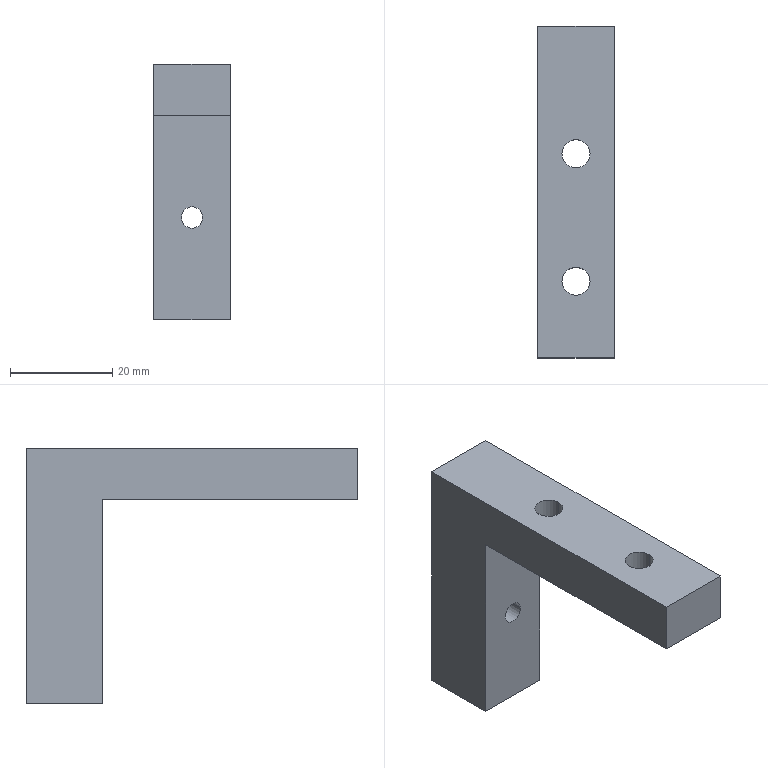Component | SolidWorks | CS021-A10-A025-1 | 1 solid | 14 faces | box 15 x 65 x 50 mm | volume 18067 mm3 | plane 8 | cylinder 6 | commonest cylinder face diameters 5.5 x4 4.2 x2 | material AL6061
build123d program:
from build123d import *

# Parameters (mm, degrees)
BOSS_EXTRUDE1_DEPTH        = 7.5
F_5_5_5_5_DIAMETER_HOLE1_D = 5.5
M5_TAPPED_HOLE1_D          = 4.2


with BuildPart() as part:
    # Sketch1 → Boss-Extrude1 (new, symmetric)
    with BuildSketch(Plane.XY):
        Polygon((10, 0), (10, 50), (50, 50), (50, 65), (0, 65), (0, 0), align=None)
    extrude(amount=BOSS_EXTRUDE1_DEPTH, both=True)

    # 5.5 _5.5_ Diameter Hole1 (through all)
    with Locations(Plane(origin=(10, 0, 0), x_dir=(0, 0, -1), z_dir=(1, 0, 0))):
        with Locations((0, 40), (0, 15)):
            Hole(F_5_5_5_5_DIAMETER_HOLE1_D / 2)

    # M5 Tapped Hole1 (through all)
    with Locations(Plane(origin=(0, 65, 0), x_dir=(1, 0, 0), z_dir=(0, 1, 0))):
        with Locations((30, 0)):
            Hole(M5_TAPPED_HOLE1_D / 2)


solid = part.part

# Placed as in the assembly
solid = solid.moved(Location((228.449, 29.817, -55), (0, 90, 0)))
STEP:
#1=CARTESIAN_POINT('',(8.911,3.142,-3.346));
#2=VERTEX_POINT('',#1);
#3=CARTESIAN_POINT('',(9.077,3.142,-3.346));
#4=VERTEX_POINT('',#3);
#5=CARTESIAN_POINT('',(8.994,3.142,-3.346));
#6=DIRECTION('',(-0.,1.,0.));
#7=DIRECTION('',(1.,0.,0.));
#8=AXIS2_PLACEMENT_3D('',#5,#6,#7);
#9=CIRCLE('',#8,0.08268);
#10=EDGE_CURVE('',#2,#4,#9,.T.);
#11=ORIENTED_EDGE('',*,*,#10,.F.);
#12=CARTESIAN_POINT('',(8.911,3.733,-3.346));
#13=VERTEX_POINT('',#12);
#14=CARTESIAN_POINT('',(8.911,3.733,-3.346));
#15=DIRECTION('',(-0.,1.,0.));
#16=VECTOR('',#15,39.37);
#17=LINE('',#14,#16);
#18=EDGE_CURVE('',#2,#13,#17,.T.);
#19=ORIENTED_EDGE('',*,*,#18,.T.);
#20=CARTESIAN_POINT('',(9.077,3.733,-3.346));
#21=VERTEX_POINT('',#20);
#22=CARTESIAN_POINT('',(8.994,3.733,-3.346));
#23=DIRECTION('',(-0.,1.,0.));
#24=DIRECTION('',(1.,0.,0.));
#25=AXIS2_PLACEMENT_3D('',#22,#23,#24);
#26=CIRCLE('',#25,0.08268);
#27=EDGE_CURVE('',#13,#21,#26,.T.);
#28=ORIENTED_EDGE('',*,*,#27,.T.);
#29=CARTESIAN_POINT('',(9.077,3.733,-3.346));
#30=DIRECTION('',(-0.,1.,0.));
#31=VECTOR('',#30,39.37);
#32=LINE('',#29,#31);
#33=EDGE_CURVE('',#4,#21,#32,.T.);
#34=ORIENTED_EDGE('',*,*,#33,.F.);
#35=EDGE_LOOP('',(#11,#19,#28,#34));
#36=FACE_OUTER_BOUND('',#35,.T.);
#37=CARTESIAN_POINT('',(8.994,3.733,-3.346));
#38=DIRECTION('',(-0.,1.,0.));
#39=DIRECTION('',(1.,0.,0.));
#40=AXIS2_PLACEMENT_3D('',#37,#38,#39);
#41=CYLINDRICAL_SURFACE('',#40,0.08268);
#42=ADVANCED_FACE('',(#36),#41,.F.);
#43=CARTESIAN_POINT('',(9.102,2.749,-2.165));
#44=VERTEX_POINT('',#43);
#45=CARTESIAN_POINT('',(8.886,2.749,-2.165));
#46=VERTEX_POINT('',#45);
#47=CARTESIAN_POINT('',(8.994,2.749,-2.165));
#48=DIRECTION('',(-0.,0.,-1.));
#49=DIRECTION('',(-1.,0.,0.));
#50=AXIS2_PLACEMENT_3D('',#47,#48,#49);
#51=CIRCLE('',#50,0.1083);
#52=EDGE_CURVE('',#44,#46,#51,.T.);
#53=ORIENTED_EDGE('',*,*,#52,.F.);
#54=CARTESIAN_POINT('',(9.102,2.749,-2.559));
#55=VERTEX_POINT('',#54);
#56=CARTESIAN_POINT('',(9.102,2.749,-2.559));
#57=DIRECTION('',(-0.,0.,-1.));
#58=VECTOR('',#57,39.37);
#59=LINE('',#56,#58);
#60=EDGE_CURVE('',#44,#55,#59,.T.);
#61=ORIENTED_EDGE('',*,*,#60,.T.);
#62=CARTESIAN_POINT('',(8.886,2.749,-2.559));
#63=VERTEX_POINT('',#62);
#64=CARTESIAN_POINT('',(8.994,2.749,-2.559));
#65=DIRECTION('',(-0.,0.,-1.));
#66=DIRECTION('',(-1.,0.,0.));
#67=AXIS2_PLACEMENT_3D('',#64,#65,#66);
#68=CIRCLE('',#67,0.1083);
#69=EDGE_CURVE('',#55,#63,#68,.T.);
#70=ORIENTED_EDGE('',*,*,#69,.T.);
#71=CARTESIAN_POINT('',(8.886,2.749,-2.559));
#72=DIRECTION('',(-0.,0.,-1.));
#73=VECTOR('',#72,39.37);
#74=LINE('',#71,#73);
#75=EDGE_CURVE('',#46,#63,#74,.T.);
#76=ORIENTED_EDGE('',*,*,#75,.F.);
#77=EDGE_LOOP('',(#53,#61,#70,#76));
#78=FACE_OUTER_BOUND('',#77,.T.);
#79=CARTESIAN_POINT('',(8.994,2.749,-2.559));
#80=DIRECTION('',(-0.,0.,-1.));
#81=DIRECTION('',(-1.,0.,0.));
#82=AXIS2_PLACEMENT_3D('',#79,#80,#81);
#83=CYLINDRICAL_SURFACE('',#82,0.1083);
#84=ADVANCED_FACE('',(#78),#83,.F.);
#85=CARTESIAN_POINT('',(9.102,1.764,-2.165));
#86=VERTEX_POINT('',#85);
#87=CARTESIAN_POINT('',(8.886,1.764,-2.165));
#88=VERTEX_POINT('',#87);
#89=CARTESIAN_POINT('',(8.994,1.764,-2.165));
#90=DIRECTION('',(-0.,0.,-1.));
#91=DIRECTION('',(-1.,0.,0.));
#92=AXIS2_PLACEMENT_3D('',#89,#90,#91);
#93=CIRCLE('',#92,0.1083);
#94=EDGE_CURVE('',#86,#88,#93,.T.);
#95=ORIENTED_EDGE('',*,*,#94,.F.);
#96=CARTESIAN_POINT('',(9.102,1.764,-2.559));
#97=VERTEX_POINT('',#96);
#98=CARTESIAN_POINT('',(9.102,1.764,-2.559));
#99=DIRECTION('',(-0.,0.,-1.));
#100=VECTOR('',#99,39.37);
#101=LINE('',#98,#100);
#102=EDGE_CURVE('',#86,#97,#101,.T.);
#103=ORIENTED_EDGE('',*,*,#102,.T.);
#104=CARTESIAN_POINT('',(8.886,1.764,-2.559));
#105=VERTEX_POINT('',#104);
#106=CARTESIAN_POINT('',(8.994,1.764,-2.559));
#107=DIRECTION('',(-0.,0.,-1.));
#108=DIRECTION('',(-1.,0.,0.));
#109=AXIS2_PLACEMENT_3D('',#106,#107,#108);
#110=CIRCLE('',#109,0.1083);
#111=EDGE_CURVE('',#97,#105,#110,.T.);
#112=ORIENTED_EDGE('',*,*,#111,.T.);
#113=CARTESIAN_POINT('',(8.886,1.764,-2.559));
#114=DIRECTION('',(-0.,0.,-1.));
#115=VECTOR('',#114,39.37);
#116=LINE('',#113,#115);
#117=EDGE_CURVE('',#88,#105,#116,.T.);
#118=ORIENTED_EDGE('',*,*,#117,.F.);
#119=EDGE_LOOP('',(#95,#103,#112,#118));
#120=FACE_OUTER_BOUND('',#119,.T.);
#121=CARTESIAN_POINT('',(8.994,1.764,-2.559));
#122=DIRECTION('',(-0.,0.,-1.));
#123=DIRECTION('',(-1.,0.,0.));
#124=AXIS2_PLACEMENT_3D('',#121,#122,#123);
#125=CYLINDRICAL_SURFACE('',#124,0.1083);
#126=ADVANCED_FACE('',(#120),#125,.F.);
#127=CARTESIAN_POINT('',(8.699,1.174,-2.165));
#128=VERTEX_POINT('',#127);
#129=CARTESIAN_POINT('',(8.699,1.174,-2.559));
#130=VERTEX_POINT('',#129);
#131=CARTESIAN_POINT('',(8.699,1.174,-2.165));
#132=DIRECTION('',(-0.,0.,-1.));
#133=VECTOR('',#132,39.37);
#134=LINE('',#131,#133);
#135=EDGE_CURVE('',#128,#130,#134,.T.);
#136=ORIENTED_EDGE('',*,*,#135,.T.);
#137=CARTESIAN_POINT('',(9.289,1.174,-2.559));
#138=VERTEX_POINT('',#137);
#139=CARTESIAN_POINT('',(9.289,1.174,-2.559));
#140=DIRECTION('',(-1.,0.,-0.));
#141=VECTOR('',#140,39.37);
#142=LINE('',#139,#141);
#143=EDGE_CURVE('',#138,#130,#142,.T.);
#144=ORIENTED_EDGE('',*,*,#143,.F.);
#145=CARTESIAN_POINT('',(9.289,1.174,-2.165));
#146=VERTEX_POINT('',#145);
#147=CARTESIAN_POINT('',(9.289,1.174,-2.165));
#148=DIRECTION('',(-0.,0.,-1.));
#149=VECTOR('',#148,39.37);
#150=LINE('',#147,#149);
#151=EDGE_CURVE('',#146,#138,#150,.T.);
#152=ORIENTED_EDGE('',*,*,#151,.F.);
#153=CARTESIAN_POINT('',(9.289,1.174,-2.165));
#154=DIRECTION('',(-1.,0.,-0.));
#155=VECTOR('',#154,39.37);
#156=LINE('',#153,#155);
#157=EDGE_CURVE('',#146,#128,#156,.T.);
#158=ORIENTED_EDGE('',*,*,#157,.T.);
#159=EDGE_LOOP('',(#136,#144,#152,#158));
#160=FACE_OUTER_BOUND('',#159,.T.);
#161=CARTESIAN_POINT('',(9.289,1.174,-2.165));
#162=DIRECTION('',(0.,1.,0.));
#163=DIRECTION('',(1.,-0.,0.));
#164=AXIS2_PLACEMENT_3D('',#161,#162,#163);
#165=PLANE('',#164);
#166=ADVANCED_FACE('',(#160),#165,.F.);
#167=CARTESIAN_POINT('',(8.994,2.749,-2.559));
#168=DIRECTION('',(-0.,0.,-1.));
#169=DIRECTION('',(-1.,0.,0.));
#170=AXIS2_PLACEMENT_3D('',#167,#168,#169);
#171=CIRCLE('',#170,0.1083);
#172=EDGE_CURVE('',#63,#55,#171,.T.);
#173=ORIENTED_EDGE('',*,*,#172,.F.);
#174=ORIENTED_EDGE('',*,*,#69,.F.);
#175=EDGE_LOOP('',(#173,#174));
#176=FACE_BOUND('',#175,.T.);
#177=CARTESIAN_POINT('',(8.994,1.764,-2.559));
#178=DIRECTION('',(-0.,0.,-1.));
#179=DIRECTION('',(-1.,0.,0.));
#180=AXIS2_PLACEMENT_3D('',#177,#178,#179);
#181=CIRCLE('',#180,0.1083);
#182=EDGE_CURVE('',#105,#97,#181,.T.);
#183=ORIENTED_EDGE('',*,*,#182,.F.);
#184=ORIENTED_EDGE('',*,*,#111,.F.);
#185=EDGE_LOOP('',(#183,#184));
#186=FACE_BOUND('',#185,.T.);
#187=CARTESIAN_POINT('',(8.699,3.142,-2.559));
#188=VERTEX_POINT('',#187);
#189=CARTESIAN_POINT('',(8.699,1.174,-2.559));
#190=DIRECTION('',(-0.,1.,0.));
#191=VECTOR('',#190,39.37);
#192=LINE('',#189,#191);
#193=EDGE_CURVE('',#130,#188,#192,.T.);
#194=ORIENTED_EDGE('',*,*,#193,.T.);
#195=CARTESIAN_POINT('',(9.289,3.142,-2.559));
#196=VERTEX_POINT('',#195);
#197=CARTESIAN_POINT('',(9.289,3.142,-2.559));
#198=DIRECTION('',(-1.,0.,-0.));
#199=VECTOR('',#198,39.37);
#200=LINE('',#197,#199);
#201=EDGE_CURVE('',#196,#188,#200,.T.);
#202=ORIENTED_EDGE('',*,*,#201,.F.);
#203=CARTESIAN_POINT('',(9.289,1.174,-2.559));
#204=DIRECTION('',(-0.,1.,0.));
#205=VECTOR('',#204,39.37);
#206=LINE('',#203,#205);
#207=EDGE_CURVE('',#138,#196,#206,.T.);
#208=ORIENTED_EDGE('',*,*,#207,.F.);
#209=ORIENTED_EDGE('',*,*,#143,.T.);
#210=EDGE_LOOP('',(#194,#202,#208,#209));
#211=FACE_OUTER_BOUND('',#210,.T.);
#212=CARTESIAN_POINT('',(9.289,1.174,-2.559));
#213=DIRECTION('',(0.,-0.,1.));
#214=DIRECTION('',(0.,-1.,-0.));
#215=AXIS2_PLACEMENT_3D('',#212,#213,#214);
#216=PLANE('',#215);
#217=ADVANCED_FACE('',(#176,#186,#211),#216,.F.);
#218=CARTESIAN_POINT('',(8.994,3.142,-3.346));
#219=DIRECTION('',(-0.,1.,0.));
#220=DIRECTION('',(1.,0.,0.));
#221=AXIS2_PLACEMENT_3D('',#218,#219,#220);
#222=CIRCLE('',#221,0.08268);
#223=EDGE_CURVE('',#4,#2,#222,.T.);
#224=ORIENTED_EDGE('',*,*,#223,.T.);
#225=ORIENTED_EDGE('',*,*,#10,.T.);
#226=EDGE_LOOP('',(#224,#225));
#227=FACE_BOUND('',#226,.T.);
#228=CARTESIAN_POINT('',(8.699,3.142,-4.134));
#229=VERTEX_POINT('',#228);
#230=CARTESIAN_POINT('',(8.699,3.142,-2.559));
#231=DIRECTION('',(-0.,0.,-1.));
#232=VECTOR('',#231,39.37);
#233=LINE('',#230,#232);
#234=EDGE_CURVE('',#188,#229,#233,.T.);
#235=ORIENTED_EDGE('',*,*,#234,.T.);
#236=CARTESIAN_POINT('',(9.289,3.142,-4.134));
#237=VERTEX_POINT('',#236);
#238=CARTESIAN_POINT('',(9.289,3.142,-4.134));
#239=DIRECTION('',(-1.,0.,-0.));
#240=VECTOR('',#239,39.37);
#241=LINE('',#238,#240);
#242=EDGE_CURVE('',#237,#229,#241,.T.);
#243=ORIENTED_EDGE('',*,*,#242,.F.);
#244=CARTESIAN_POINT('',(9.289,3.142,-2.559));
#245=DIRECTION('',(-0.,0.,-1.));
#246=VECTOR('',#245,39.37);
#247=LINE('',#244,#246);
#248=EDGE_CURVE('',#196,#237,#247,.T.);
#249=ORIENTED_EDGE('',*,*,#248,.F.);
#250=ORIENTED_EDGE('',*,*,#201,.T.);
#251=EDGE_LOOP('',(#235,#243,#249,#250));
#252=FACE_OUTER_BOUND('',#251,.T.);
#253=CARTESIAN_POINT('',(9.289,3.142,-2.559));
#254=DIRECTION('',(0.,1.,0.));
#255=DIRECTION('',(1.,-0.,0.));
#256=AXIS2_PLACEMENT_3D('',#253,#254,#255);
#257=PLANE('',#256);
#258=ADVANCED_FACE('',(#227,#252),#257,.F.);
#259=CARTESIAN_POINT('',(8.699,3.733,-4.134));
#260=VERTEX_POINT('',#259);
#261=CARTESIAN_POINT('',(8.699,3.142,-4.134));
#262=DIRECTION('',(-0.,1.,0.));
#263=VECTOR('',#262,39.37);
#264=LINE('',#261,#263);
#265=EDGE_CURVE('',#229,#260,#264,.T.);
#266=ORIENTED_EDGE('',*,*,#265,.T.);
#267=CARTESIAN_POINT('',(9.289,3.733,-4.134));
#268=VERTEX_POINT('',#267);
#269=CARTESIAN_POINT('',(9.289,3.733,-4.134));
#270=DIRECTION('',(-1.,0.,-0.));
#271=VECTOR('',#270,39.37);
#272=LINE('',#269,#271);
#273=EDGE_CURVE('',#268,#260,#272,.T.);
#274=ORIENTED_EDGE('',*,*,#273,.F.);
#275=CARTESIAN_POINT('',(9.289,3.142,-4.134));
#276=DIRECTION('',(-0.,1.,0.));
#277=VECTOR('',#276,39.37);
#278=LINE('',#275,#277);
#279=EDGE_CURVE('',#237,#268,#278,.T.);
#280=ORIENTED_EDGE('',*,*,#279,.F.);
#281=ORIENTED_EDGE('',*,*,#242,.T.);
#282=EDGE_LOOP('',(#266,#274,#280,#281));
#283=FACE_OUTER_BOUND('',#282,.T.);
#284=CARTESIAN_POINT('',(9.289,3.142,-4.134));
#285=DIRECTION('',(-0.,-0.,1.));
#286=DIRECTION('',(1.,-0.,0.));
#287=AXIS2_PLACEMENT_3D('',#284,#285,#286);
#288=PLANE('',#287);
#289=ADVANCED_FACE('',(#283),#288,.F.);
#290=CARTESIAN_POINT('',(8.994,3.733,-3.346));
#291=DIRECTION('',(-0.,1.,0.));
#292=DIRECTION('',(1.,0.,0.));
#293=AXIS2_PLACEMENT_3D('',#290,#291,#292);
#294=CIRCLE('',#293,0.08268);
#295=EDGE_CURVE('',#21,#13,#294,.T.);
#296=ORIENTED_EDGE('',*,*,#295,.F.);
#297=ORIENTED_EDGE('',*,*,#27,.F.);
#298=EDGE_LOOP('',(#296,#297));
#299=FACE_BOUND('',#298,.T.);
#300=CARTESIAN_POINT('',(8.699,3.733,-2.165));
#301=VERTEX_POINT('',#300);
#302=CARTESIAN_POINT('',(8.699,3.733,-2.165));
#303=DIRECTION('',(-0.,0.,-1.));
#304=VECTOR('',#303,39.37);
#305=LINE('',#302,#304);
#306=EDGE_CURVE('',#301,#260,#305,.T.);
#307=ORIENTED_EDGE('',*,*,#306,.F.);
#308=CARTESIAN_POINT('',(9.289,3.733,-2.165));
#309=VERTEX_POINT('',#308);
#310=CARTESIAN_POINT('',(9.289,3.733,-2.165));
#311=DIRECTION('',(-1.,0.,-0.));
#312=VECTOR('',#311,39.37);
#313=LINE('',#310,#312);
#314=EDGE_CURVE('',#309,#301,#313,.T.);
#315=ORIENTED_EDGE('',*,*,#314,.F.);
#316=CARTESIAN_POINT('',(9.289,3.733,-2.165));
#317=DIRECTION('',(-0.,0.,-1.));
#318=VECTOR('',#317,39.37);
#319=LINE('',#316,#318);
#320=EDGE_CURVE('',#309,#268,#319,.T.);
#321=ORIENTED_EDGE('',*,*,#320,.T.);
#322=ORIENTED_EDGE('',*,*,#273,.T.);
#323=EDGE_LOOP('',(#307,#315,#321,#322));
#324=FACE_OUTER_BOUND('',#323,.T.);
#325=CARTESIAN_POINT('',(9.289,3.733,-2.165));
#326=DIRECTION('',(0.,1.,0.));
#327=DIRECTION('',(1.,-0.,0.));
#328=AXIS2_PLACEMENT_3D('',#325,#326,#327);
#329=PLANE('',#328);
#330=ADVANCED_FACE('',(#299,#324),#329,.T.);
#331=CARTESIAN_POINT('',(8.994,2.749,-2.165));
#332=DIRECTION('',(-0.,0.,-1.));
#333=DIRECTION('',(-1.,0.,0.));
#334=AXIS2_PLACEMENT_3D('',#331,#332,#333);
#335=CIRCLE('',#334,0.1083);
#336=EDGE_CURVE('',#46,#44,#335,.T.);
#337=ORIENTED_EDGE('',*,*,#336,.T.);
#338=ORIENTED_EDGE('',*,*,#52,.T.);
#339=EDGE_LOOP('',(#337,#338));
#340=FACE_BOUND('',#339,.T.);
#341=CARTESIAN_POINT('',(8.994,1.764,-2.165));
#342=DIRECTION('',(-0.,0.,-1.));
#343=DIRECTION('',(-1.,0.,0.));
#344=AXIS2_PLACEMENT_3D('',#341,#342,#343);
#345=CIRCLE('',#344,0.1083);
#346=EDGE_CURVE('',#88,#86,#345,.T.);
#347=ORIENTED_EDGE('',*,*,#346,.T.);
#348=ORIENTED_EDGE('',*,*,#94,.T.);
#349=EDGE_LOOP('',(#347,#348));
#350=FACE_BOUND('',#349,.T.);
#351=CARTESIAN_POINT('',(8.699,1.174,-2.165));
#352=DIRECTION('',(-0.,1.,0.));
#353=VECTOR('',#352,39.37);
#354=LINE('',#351,#353);
#355=EDGE_CURVE('',#128,#301,#354,.T.);
#356=ORIENTED_EDGE('',*,*,#355,.F.);
#357=ORIENTED_EDGE('',*,*,#157,.F.);
#358=CARTESIAN_POINT('',(9.289,1.174,-2.165));
#359=DIRECTION('',(-0.,1.,0.));
#360=VECTOR('',#359,39.37);
#361=LINE('',#358,#360);
#362=EDGE_CURVE('',#146,#309,#361,.T.);
#363=ORIENTED_EDGE('',*,*,#362,.T.);
#364=ORIENTED_EDGE('',*,*,#314,.T.);
#365=EDGE_LOOP('',(#356,#357,#363,#364));
#366=FACE_OUTER_BOUND('',#365,.T.);
#367=CARTESIAN_POINT('',(9.289,1.174,-2.165));
#368=DIRECTION('',(-0.,-0.,1.));
#369=DIRECTION('',(1.,-0.,0.));
#370=AXIS2_PLACEMENT_3D('',#367,#368,#369);
#371=PLANE('',#370);
#372=ADVANCED_FACE('',(#340,#350,#366),#371,.T.);
#373=ORIENTED_EDGE('',*,*,#151,.T.);
#374=ORIENTED_EDGE('',*,*,#207,.T.);
#375=ORIENTED_EDGE('',*,*,#248,.T.);
#376=ORIENTED_EDGE('',*,*,#279,.T.);
#377=ORIENTED_EDGE('',*,*,#320,.F.);
#378=ORIENTED_EDGE('',*,*,#362,.F.);
#379=EDGE_LOOP('',(#373,#374,#375,#376,#377,#378));
#380=FACE_OUTER_BOUND('',#379,.T.);
#381=CARTESIAN_POINT('',(9.289,1.174,-2.165));
#382=DIRECTION('',(1.,-0.,-0.));
#383=DIRECTION('',(-0.,0.,-1.));
#384=AXIS2_PLACEMENT_3D('',#381,#382,#383);
#385=PLANE('',#384);
#386=ADVANCED_FACE('',(#380),#385,.T.);
#387=ORIENTED_EDGE('',*,*,#135,.F.);
#388=ORIENTED_EDGE('',*,*,#355,.T.);
#389=ORIENTED_EDGE('',*,*,#306,.T.);
#390=ORIENTED_EDGE('',*,*,#265,.F.);
#391=ORIENTED_EDGE('',*,*,#234,.F.);
#392=ORIENTED_EDGE('',*,*,#193,.F.);
#393=EDGE_LOOP('',(#387,#388,#389,#390,#391,#392));
#394=FACE_OUTER_BOUND('',#393,.T.);
#395=CARTESIAN_POINT('',(8.699,1.174,-2.165));
#396=DIRECTION('',(1.,-0.,-0.));
#397=DIRECTION('',(-0.,0.,-1.));
#398=AXIS2_PLACEMENT_3D('',#395,#396,#397);
#399=PLANE('',#398);
#400=ADVANCED_FACE('',(#394),#399,.F.);
#401=ORIENTED_EDGE('',*,*,#102,.F.);
#402=ORIENTED_EDGE('',*,*,#346,.F.);
#403=ORIENTED_EDGE('',*,*,#117,.T.);
#404=ORIENTED_EDGE('',*,*,#182,.T.);
#405=EDGE_LOOP('',(#401,#402,#403,#404));
#406=FACE_OUTER_BOUND('',#405,.T.);
#407=CARTESIAN_POINT('',(8.994,1.764,-2.559));
#408=DIRECTION('',(-0.,0.,-1.));
#409=DIRECTION('',(-1.,0.,0.));
#410=AXIS2_PLACEMENT_3D('',#407,#408,#409);
#411=CYLINDRICAL_SURFACE('',#410,0.1083);
#412=ADVANCED_FACE('',(#406),#411,.F.);
#413=ORIENTED_EDGE('',*,*,#60,.F.);
#414=ORIENTED_EDGE('',*,*,#336,.F.);
#415=ORIENTED_EDGE('',*,*,#75,.T.);
#416=ORIENTED_EDGE('',*,*,#172,.T.);
#417=EDGE_LOOP('',(#413,#414,#415,#416));
#418=FACE_OUTER_BOUND('',#417,.T.);
#419=CARTESIAN_POINT('',(8.994,2.749,-2.559));
#420=DIRECTION('',(-0.,0.,-1.));
#421=DIRECTION('',(-1.,0.,0.));
#422=AXIS2_PLACEMENT_3D('',#419,#420,#421);
#423=CYLINDRICAL_SURFACE('',#422,0.1083);
#424=ADVANCED_FACE('',(#418),#423,.F.);
#425=ORIENTED_EDGE('',*,*,#18,.F.);
#426=ORIENTED_EDGE('',*,*,#223,.F.);
#427=ORIENTED_EDGE('',*,*,#33,.T.);
#428=ORIENTED_EDGE('',*,*,#295,.T.);
#429=EDGE_LOOP('',(#425,#426,#427,#428));
#430=FACE_OUTER_BOUND('',#429,.T.);
#431=CARTESIAN_POINT('',(8.994,3.733,-3.346));
#432=DIRECTION('',(-0.,1.,0.));
#433=DIRECTION('',(1.,0.,0.));
#434=AXIS2_PLACEMENT_3D('',#431,#432,#433);
#435=CYLINDRICAL_SURFACE('',#434,0.08268);
#436=ADVANCED_FACE('',(#430),#435,.F.);
#437=CLOSED_SHELL('',(#42,#84,#126,#166,#217,#258,#289,#330,#372,#386,#400,#412,#424,#436));
#438=MANIFOLD_SOLID_BREP('',#437);
#439=CARTESIAN_POINT('',(0.,0.,0.));
#440=DIRECTION('',(0.,0.,1.));
#441=DIRECTION('',(1.,0.,0.));
#442=AXIS2_PLACEMENT_3D('',#439,#440,#441);
#443=(LENGTH_UNIT()NAMED_UNIT(*)SI_UNIT($,.METRE.));
#444=LENGTH_MEASURE_WITH_UNIT(LENGTH_MEASURE(0.0254),#443);
#445=DIMENSIONAL_EXPONENTS(1.,0.,0.,0.,0.,0.,0.);
#446=(CONVERSION_BASED_UNIT('',#444)LENGTH_UNIT()NAMED_UNIT(#445));
#447=UNCERTAINTY_MEASURE_WITH_UNIT(LENGTH_MEASURE(0.00001),#446,'','');
#448=(NAMED_UNIT(*)PLANE_ANGLE_UNIT()SI_UNIT($,.RADIAN.));
#449=(NAMED_UNIT(*)SI_UNIT($,.STERADIAN.)SOLID_ANGLE_UNIT());
#450=(GEOMETRIC_REPRESENTATION_CONTEXT(3)GLOBAL_UNCERTAINTY_ASSIGNED_CONTEXT((#447))GLOBAL_UNIT_ASSIGNED_CONTEXT((#446,#448,#449))REPRESENTATION_CONTEXT('',''));
#451=ADVANCED_BREP_SHAPE_REPRESENTATION('',(#438,#442),#450);
#452=COLOUR_RGB('',0.7922,0.8196,0.9333);
#453=FILL_AREA_STYLE_COLOUR('',#452);
#454=FILL_AREA_STYLE('',(#453));
#455=SURFACE_STYLE_FILL_AREA(#454);
#456=SURFACE_SIDE_STYLE('',(#455));
#457=SURFACE_STYLE_USAGE(.BOTH.,#456);
#458=PRESENTATION_STYLE_ASSIGNMENT((#457));
#459=STYLED_ITEM('',(#458),#438);
#460=PRESENTATION_LAYER_ASSIGNMENT('','',(#459));
#461=(LENGTH_UNIT()NAMED_UNIT(*)SI_UNIT($,.METRE.));
#462=LENGTH_MEASURE_WITH_UNIT(LENGTH_MEASURE(0.0254),#461);
#463=DIMENSIONAL_EXPONENTS(1.,0.,0.,0.,0.,0.,0.);
#464=(CONVERSION_BASED_UNIT('',#462)LENGTH_UNIT()NAMED_UNIT(#463));
#465=UNCERTAINTY_MEASURE_WITH_UNIT(LENGTH_MEASURE(0.00001),#464,'','');
#466=(NAMED_UNIT(*)PLANE_ANGLE_UNIT()SI_UNIT($,.RADIAN.));
#467=(NAMED_UNIT(*)SI_UNIT($,.STERADIAN.)SOLID_ANGLE_UNIT());
#468=(GEOMETRIC_REPRESENTATION_CONTEXT(3)GLOBAL_UNCERTAINTY_ASSIGNED_CONTEXT((#465))GLOBAL_UNIT_ASSIGNED_CONTEXT((#464,#466,#467))REPRESENTATION_CONTEXT('',''));
#469=MECHANICAL_DESIGN_GEOMETRIC_PRESENTATION_REPRESENTATION('',(#459),#468);